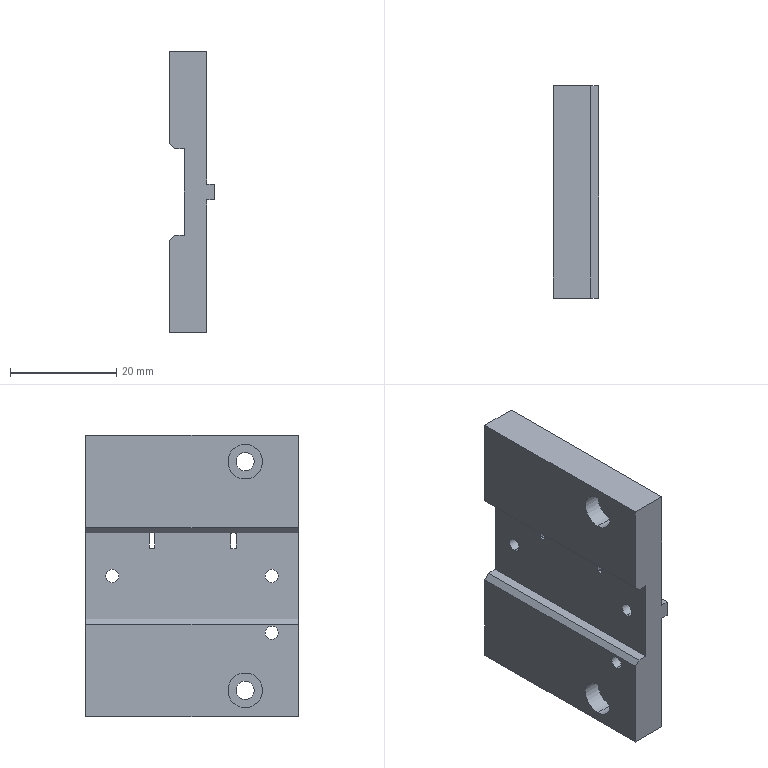Component | SolidWorks | 7.1.02.0001.00.00-0082-1 | 1 solid | 46 faces | box 8.5 x 40 x 53 mm | volume 12759 mm3 | plane 24 | cylinder 22 | commonest cylinder face diameters 0.3 x8 2.5 x6 6.5 x4 3.4 x4
build123d program:
from build123d import *

# Parameters (mm, degrees)
SKETCH1_W                                       = 53
SKETCH1_H                                       = 40
BOSS_EXTRUDE1_DEPTH                             = 7
M3_HEX_SOCKET_HEAD_CAP_SCREW_CBORE1_D           = 3.4
M3_HEX_SOCKET_HEAD_CAP_SCREW_CBORE1_CBORE_D     = 6.5
M3_HEX_SOCKET_HEAD_CAP_SCREW_CBORE1_CBORE_DEPTH = 3.4
SKETCH3_W                                       = 3
SKETCH3_H                                       = 1.5
BOSS_EXTRUDE2_DEPTH                             = 40
SKETCH4_W                                       = 16.2
SKETCH4_H                                       = 2.8
CUT_EXTRUDE1_DEPTH                              = 49.49
CHAMFER1_SIZE                                   = 1
M3X0_5_TAPPED_HOLE1_D                           = 2.5
SKETCH6_W                                       = 3
SKETCH6_H                                       = 1
CUT_EXTRUDE2_DEPTH                              = 35.271
FILLET1_R                                       = 0.15
M3X0_5_TAPPED_HOLE2_D                           = 2.5


with BuildPart() as part:
    # Sketch1 → Boss-Extrude1 (new body)
    with BuildSketch(Plane.XY):
        Rectangle(SKETCH1_W, SKETCH1_H)
    extrude(amount=BOSS_EXTRUDE1_DEPTH)

    # M3 Hex Socket Head Cap Screw CBORE1 (through all)
    with Locations(Plane(origin=(21.5, -10, 7), x_dir=(1, 0, 0), z_dir=(0, 0, 1))):
        with Locations((0, 0), (-43, 0)):
            CounterBoreHole(M3_HEX_SOCKET_HEAD_CAP_SCREW_CBORE1_D / 2, M3_HEX_SOCKET_HEAD_CAP_SCREW_CBORE1_CBORE_D / 2, M3_HEX_SOCKET_HEAD_CAP_SCREW_CBORE1_CBORE_DEPTH)

    # Sketch3 → Boss-Extrude2 (add)
    with BuildSketch(Plane.XZ.offset(20)):
        with Locations((0, -0.75)):
            Rectangle(SKETCH3_W, SKETCH3_H)
    extrude(amount=-BOSS_EXTRUDE2_DEPTH)

    # Sketch4 → Cut-Extrude1 (cut, through all)
    with BuildSketch(Plane.XZ.offset(20)):
        with Locations((0, 5.6)):
            Rectangle(SKETCH4_W, SKETCH4_H)
    extrude(amount=-CUT_EXTRUDE1_DEPTH, mode=Mode.SUBTRACT)

    # Chamfer1
    chamfer1_edges = [part.edges().sort_by_distance(p)[0] for p in [
        (8.1, 0, 7),
        (-8.1, 0, 7),
    ]]
    chamfer(chamfer1_edges, length=CHAMFER1_SIZE)

    # M3x0.5 Tapped Hole1 (through all)
    with Locations(Plane(origin=(0, -15, 4.2), x_dir=(1, 0, 0), z_dir=(0, 0, 1))):
        with Locations((0, 0), (0, 30)):
            Hole(M3X0_5_TAPPED_HOLE1_D / 2)

    # Sketch6 → Cut-Extrude2 (cut, through all)
    with BuildSketch(Plane.XY.offset(7)):
        with Locations((6.6, -7.8)):
            Rectangle(SKETCH6_W, SKETCH6_H)
        with Locations((6.6, 7.5)):
            Rectangle(SKETCH6_W, SKETCH6_H)
    extrude(amount=-CUT_EXTRUDE2_DEPTH, mode=Mode.SUBTRACT)

    # Fillet1
    fillet1_edges = [part.edges().sort_by_distance(p)[0] for p in [
        (5.1, 7, 2.1),
        (5.1, 8, 2.1),
        (8.1, 7, 2.1),
        (8.1, 8, 2.1),
        (5.1, -8.3, 2.1),
        (5.1, -7.3, 2.1),
        (8.1, -8.3, 2.1),
        (8.1, -7.3, 2.1),
    ]]
    fillet(fillet1_edges, radius=FILLET1_R)

    # M3x0.5 Tapped Hole2 (through all)
    with Locations(Plane(origin=(-10.7, -15, 7), x_dir=(1, 0, 0), z_dir=(0, 0, 1))):
        with Locations((0, 0)):
            Hole(M3X0_5_TAPPED_HOLE2_D / 2)


solid = part.part

# Placed as in the assembly
solid = solid.moved(Location((-60.964, 23.316, 0), (0, -90, 0)))